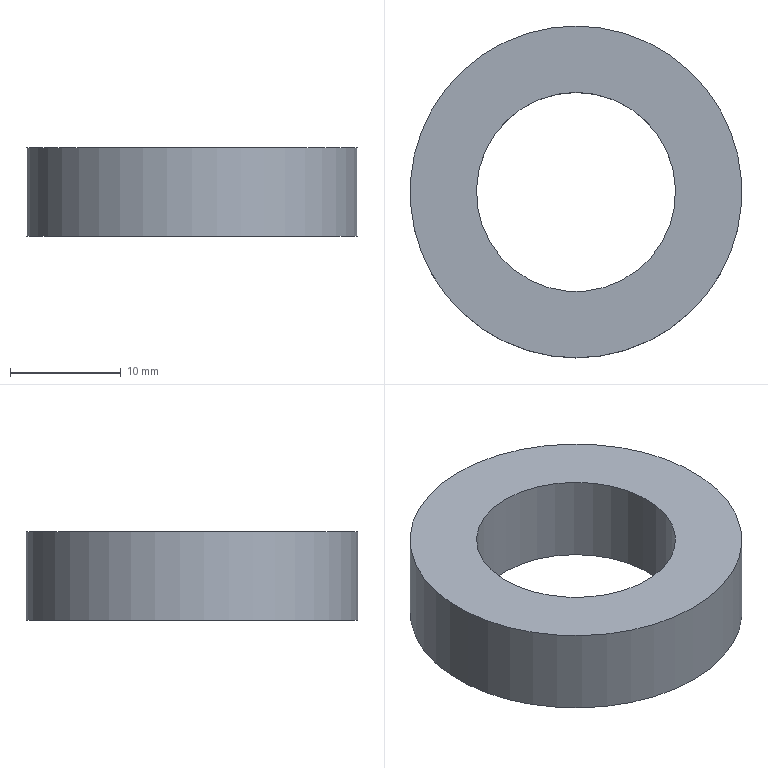Component | NX | 15 | 1 solid | 8 faces | box 30 x 30 x 8 mm | volume 2262 mm3 | plane 4 | cylinder 4 | commonest cylinder face diameters 30 x1 18 x1 21 x1 27 x1
STEP:
#1=CARTESIAN_POINT('',(0.,0.,0.));
#2=DIRECTION('',(0.,0.,1.));
#3=DIRECTION('',(1.,0.,0.));
#4=AXIS2_PLACEMENT_3D('',#1,#2,#3);
#5=CARTESIAN_POINT('',(0.,31.5,-46.));
#6=VERTEX_POINT('',#5);
#7=CARTESIAN_POINT('',(0.,16.5,-46.));
#8=DIRECTION('',(0.,0.,-1.));
#9=DIRECTION('',(0.,1.,0.));
#10=AXIS2_PLACEMENT_3D('',#7,#8,#9);
#11=CIRCLE('',#10,15.);
#12=CARTESIAN_POINT('',(0.,30.,-46.));
#13=DIRECTION('',(0.,0.,-1.));
#14=DIRECTION('',(0.,1.,0.));
#15=AXIS2_PLACEMENT_3D('',#12,#13,#14);
#16=PLANE('',#15);
#17=CARTESIAN_POINT('',(-13.5,0.));
#18=DIRECTION('',(1.,0.));
#19=AXIS2_PLACEMENT_2D('',#17,#18);
#20=CIRCLE('',#19,15.);
#21=(GEOMETRIC_REPRESENTATION_CONTEXT(2)PARAMETRIC_REPRESENTATION_CONTEXT()REPRESENTATION_CONTEXT('',''));
#22=DEFINITIONAL_REPRESENTATION('',(#20),#21);
#23=PCURVE('',#16,#22);
#24=CARTESIAN_POINT('',(0.,16.5,-46.));
#25=DIRECTION('',(0.,0.,-1.));
#26=DIRECTION('',(0.,1.,0.));
#27=AXIS2_PLACEMENT_3D('',#24,#25,#26);
#28=CYLINDRICAL_SURFACE('',#27,15.);
#29=CARTESIAN_POINT('',(0.,0.));
#30=DIRECTION('',(1.,0.));
#31=VECTOR('',#30,1.);
#32=LINE('',#29,#31);
#33=(GEOMETRIC_REPRESENTATION_CONTEXT(2)PARAMETRIC_REPRESENTATION_CONTEXT()REPRESENTATION_CONTEXT('',''));
#34=DEFINITIONAL_REPRESENTATION('',(#32),#33);
#35=PCURVE('',#28,#34);
#36=SURFACE_CURVE('',#11,(#23,#35),.PCURVE_S1.);
#37=EDGE_CURVE('',#6,#6,#36,.T.);
#38=ORIENTED_EDGE('',*,*,#37,.T.);
#39=EDGE_LOOP('',(#38));
#40=FACE_BOUND('',#39,.T.);
#41=CARTESIAN_POINT('',(0.,30.,-46.));
#42=VERTEX_POINT('',#41);
#43=CARTESIAN_POINT('',(0.,16.5,-46.));
#44=DIRECTION('',(0.,0.,-1.));
#45=DIRECTION('',(0.,1.,0.));
#46=AXIS2_PLACEMENT_3D('',#43,#44,#45);
#47=CIRCLE('',#46,13.5);
#48=CARTESIAN_POINT('',(-13.5,0.));
#49=DIRECTION('',(1.,0.));
#50=AXIS2_PLACEMENT_2D('',#48,#49);
#51=CIRCLE('',#50,13.5);
#52=(GEOMETRIC_REPRESENTATION_CONTEXT(2)PARAMETRIC_REPRESENTATION_CONTEXT()REPRESENTATION_CONTEXT('',''));
#53=DEFINITIONAL_REPRESENTATION('',(#51),#52);
#54=PCURVE('',#16,#53);
#55=CARTESIAN_POINT('',(0.,16.5,-46.));
#56=DIRECTION('',(0.,0.,-1.));
#57=DIRECTION('',(0.,1.,0.));
#58=AXIS2_PLACEMENT_3D('',#55,#56,#57);
#59=CYLINDRICAL_SURFACE('',#58,13.5);
#60=CARTESIAN_POINT('',(0.,0.));
#61=DIRECTION('',(1.,0.));
#62=VECTOR('',#61,1.);
#63=LINE('',#60,#62);
#64=(GEOMETRIC_REPRESENTATION_CONTEXT(2)PARAMETRIC_REPRESENTATION_CONTEXT()REPRESENTATION_CONTEXT('',''));
#65=DEFINITIONAL_REPRESENTATION('',(#63),#64);
#66=PCURVE('',#59,#65);
#67=SURFACE_CURVE('',#47,(#54,#66),.PCURVE_S1.);
#68=EDGE_CURVE('',#42,#42,#67,.T.);
#69=ORIENTED_EDGE('',*,*,#68,.F.);
#70=EDGE_LOOP('',(#69));
#71=FACE_BOUND('',#70,.T.);
#72=ADVANCED_FACE('',(#40,#71),#16,.T.);
#73=CARTESIAN_POINT('',(0.,31.5,-38.));
#74=VERTEX_POINT('',#73);
#75=CARTESIAN_POINT('',(0.,16.5,-38.));
#76=DIRECTION('',(0.,0.,-1.));
#77=DIRECTION('',(0.,1.,0.));
#78=AXIS2_PLACEMENT_3D('',#75,#76,#77);
#79=CIRCLE('',#78,15.);
#80=CARTESIAN_POINT('',(0.,-8.));
#81=DIRECTION('',(1.,0.));
#82=VECTOR('',#81,1.);
#83=LINE('',#80,#82);
#84=(GEOMETRIC_REPRESENTATION_CONTEXT(2)PARAMETRIC_REPRESENTATION_CONTEXT()REPRESENTATION_CONTEXT('',''));
#85=DEFINITIONAL_REPRESENTATION('',(#83),#84);
#86=PCURVE('',#28,#85);
#87=CARTESIAN_POINT('',(0.,31.5,-38.));
#88=DIRECTION('',(0.,0.,1.));
#89=DIRECTION('',(0.,-1.,0.));
#90=AXIS2_PLACEMENT_3D('',#87,#88,#89);
#91=PLANE('',#90);
#92=CARTESIAN_POINT('',(0.,0.));
#93=CARTESIAN_POINT('',(0.,25.981));
#94=CARTESIAN_POINT('',(22.5,12.99));
#95=CARTESIAN_POINT('',(45.,0.));
#96=CARTESIAN_POINT('',(22.5,-12.99));
#97=CARTESIAN_POINT('',(0.,-25.981));
#98=CARTESIAN_POINT('',(0.,0.));
#99=(BOUNDED_CURVE()B_SPLINE_CURVE(2,(#92,#93,#94,#95,#96,#97,#98),.UNSPECIFIED.,.T.,.F.)B_SPLINE_CURVE_WITH_KNOTS((1,2,2,2,2,1),(-2.094,0.,2.094,4.189,6.283,8.378),.UNSPECIFIED.)CURVE()GEOMETRIC_REPRESENTATION_ITEM()RATIONAL_B_SPLINE_CURVE((1.,0.5,1.,0.5,1.,0.5,1.))REPRESENTATION_ITEM(''));
#100=(GEOMETRIC_REPRESENTATION_CONTEXT(2)PARAMETRIC_REPRESENTATION_CONTEXT()REPRESENTATION_CONTEXT('',''));
#101=DEFINITIONAL_REPRESENTATION('',(#99),#100);
#102=PCURVE('',#91,#101);
#103=SURFACE_CURVE('',#79,(#86,#102),.PCURVE_S1.);
#104=EDGE_CURVE('',#74,#74,#103,.T.);
#105=ORIENTED_EDGE('',*,*,#104,.T.);
#106=CARTESIAN_POINT('',(0.,31.5,-38.));
#107=CARTESIAN_POINT('',(0.,31.5,-46.));
#108=B_SPLINE_CURVE_WITH_KNOTS('',1,(#106,#107),.UNSPECIFIED.,.F.,.F.,(2,2),(-8.,0.),.PIECEWISE_BEZIER_KNOTS.);
#109=CARTESIAN_POINT('',(6.283,0.));
#110=DIRECTION('',(0.,1.));
#111=VECTOR('',#110,1.);
#112=LINE('',#109,#111);
#113=(GEOMETRIC_REPRESENTATION_CONTEXT(2)PARAMETRIC_REPRESENTATION_CONTEXT()REPRESENTATION_CONTEXT('',''));
#114=DEFINITIONAL_REPRESENTATION('',(#112),#113);
#115=PCURVE('',#28,#114);
#116=CARTESIAN_POINT('',(0.,0.));
#117=DIRECTION('',(0.,1.));
#118=VECTOR('',#117,1.);
#119=LINE('',#116,#118);
#120=(GEOMETRIC_REPRESENTATION_CONTEXT(2)PARAMETRIC_REPRESENTATION_CONTEXT()REPRESENTATION_CONTEXT('',''));
#121=DEFINITIONAL_REPRESENTATION('',(#119),#120);
#122=PCURVE('',#28,#121);
#123=SEAM_CURVE('',#108,(#115,#122),.PCURVE_S1.);
#124=EDGE_CURVE('',#74,#6,#123,.T.);
#125=ORIENTED_EDGE('',*,*,#124,.T.);
#126=ORIENTED_EDGE('',*,*,#37,.F.);
#127=ORIENTED_EDGE('',*,*,#124,.F.);
#128=EDGE_LOOP('',(#105,#125,#126,#127));
#129=FACE_BOUND('',#128,.T.);
#130=ADVANCED_FACE('',(#129),#28,.T.);
#131=CARTESIAN_POINT('',(0.,25.5,-38.));
#132=VERTEX_POINT('',#131);
#133=CARTESIAN_POINT('',(0.,16.5,-38.));
#134=DIRECTION('',(0.,0.,-1.));
#135=DIRECTION('',(0.,1.,0.));
#136=AXIS2_PLACEMENT_3D('',#133,#134,#135);
#137=CIRCLE('',#136,9.);
#138=CARTESIAN_POINT('',(6.,0.));
#139=CARTESIAN_POINT('',(6.,15.588));
#140=CARTESIAN_POINT('',(19.5,7.794));
#141=CARTESIAN_POINT('',(33.,0.));
#142=CARTESIAN_POINT('',(19.5,-7.794));
#143=CARTESIAN_POINT('',(6.,-15.588));
#144=CARTESIAN_POINT('',(6.,0.));
#145=(BOUNDED_CURVE()B_SPLINE_CURVE(2,(#138,#139,#140,#141,#142,#143,#144),.UNSPECIFIED.,.T.,.F.)B_SPLINE_CURVE_WITH_KNOTS((1,2,2,2,2,1),(-2.094,0.,2.094,4.189,6.283,8.378),.UNSPECIFIED.)CURVE()GEOMETRIC_REPRESENTATION_ITEM()RATIONAL_B_SPLINE_CURVE((1.,0.5,1.,0.5,1.,0.5,1.))REPRESENTATION_ITEM(''));
#146=(GEOMETRIC_REPRESENTATION_CONTEXT(2)PARAMETRIC_REPRESENTATION_CONTEXT()REPRESENTATION_CONTEXT('',''));
#147=DEFINITIONAL_REPRESENTATION('',(#145),#146);
#148=PCURVE('',#91,#147);
#149=CARTESIAN_POINT('',(0.,16.5,-46.));
#150=DIRECTION('',(0.,0.,-1.));
#151=DIRECTION('',(0.,1.,0.));
#152=AXIS2_PLACEMENT_3D('',#149,#150,#151);
#153=CYLINDRICAL_SURFACE('',#152,9.);
#154=CARTESIAN_POINT('',(0.,-8.));
#155=DIRECTION('',(1.,0.));
#156=VECTOR('',#155,1.);
#157=LINE('',#154,#156);
#158=(GEOMETRIC_REPRESENTATION_CONTEXT(2)PARAMETRIC_REPRESENTATION_CONTEXT()REPRESENTATION_CONTEXT('',''));
#159=DEFINITIONAL_REPRESENTATION('',(#157),#158);
#160=PCURVE('',#153,#159);
#161=SURFACE_CURVE('',#137,(#148,#160),.PCURVE_S1.);
#162=EDGE_CURVE('',#132,#132,#161,.T.);
#163=ORIENTED_EDGE('',*,*,#162,.T.);
#164=EDGE_LOOP('',(#163));
#165=FACE_BOUND('',#164,.T.);
#166=ORIENTED_EDGE('',*,*,#104,.F.);
#167=EDGE_LOOP('',(#166));
#168=FACE_BOUND('',#167,.T.);
#169=ADVANCED_FACE('',(#165,#168),#91,.T.);
#170=CARTESIAN_POINT('',(0.,25.5,-46.));
#171=VERTEX_POINT('',#170);
#172=CARTESIAN_POINT('',(0.,16.5,-46.));
#173=DIRECTION('',(0.,0.,-1.));
#174=DIRECTION('',(0.,1.,0.));
#175=AXIS2_PLACEMENT_3D('',#172,#173,#174);
#176=CIRCLE('',#175,9.);
#177=CARTESIAN_POINT('',(0.,0.));
#178=DIRECTION('',(1.,0.));
#179=VECTOR('',#178,1.);
#180=LINE('',#177,#179);
#181=(GEOMETRIC_REPRESENTATION_CONTEXT(2)PARAMETRIC_REPRESENTATION_CONTEXT()REPRESENTATION_CONTEXT('',''));
#182=DEFINITIONAL_REPRESENTATION('',(#180),#181);
#183=PCURVE('',#153,#182);
#184=CARTESIAN_POINT('',(0.,25.5,-46.));
#185=DIRECTION('',(0.,0.,-1.));
#186=DIRECTION('',(0.,1.,0.));
#187=AXIS2_PLACEMENT_3D('',#184,#185,#186);
#188=PLANE('',#187);
#189=CARTESIAN_POINT('',(-9.,0.));
#190=DIRECTION('',(1.,0.));
#191=AXIS2_PLACEMENT_2D('',#189,#190);
#192=CIRCLE('',#191,9.);
#193=(GEOMETRIC_REPRESENTATION_CONTEXT(2)PARAMETRIC_REPRESENTATION_CONTEXT()REPRESENTATION_CONTEXT('',''));
#194=DEFINITIONAL_REPRESENTATION('',(#192),#193);
#195=PCURVE('',#188,#194);
#196=SURFACE_CURVE('',#176,(#183,#195),.PCURVE_S1.);
#197=EDGE_CURVE('',#171,#171,#196,.T.);
#198=ORIENTED_EDGE('',*,*,#197,.F.);
#199=CARTESIAN_POINT('',(-0.,25.5,-38.));
#200=CARTESIAN_POINT('',(-0.,25.5,-46.));
#201=B_SPLINE_CURVE_WITH_KNOTS('',1,(#199,#200),.UNSPECIFIED.,.F.,.F.,(2,2),(-8.,0.),.PIECEWISE_BEZIER_KNOTS.);
#202=CARTESIAN_POINT('',(0.,0.));
#203=DIRECTION('',(0.,1.));
#204=VECTOR('',#203,1.);
#205=LINE('',#202,#204);
#206=(GEOMETRIC_REPRESENTATION_CONTEXT(2)PARAMETRIC_REPRESENTATION_CONTEXT()REPRESENTATION_CONTEXT('',''));
#207=DEFINITIONAL_REPRESENTATION('',(#205),#206);
#208=PCURVE('',#153,#207);
#209=CARTESIAN_POINT('',(6.283,0.));
#210=DIRECTION('',(0.,1.));
#211=VECTOR('',#210,1.);
#212=LINE('',#209,#211);
#213=(GEOMETRIC_REPRESENTATION_CONTEXT(2)PARAMETRIC_REPRESENTATION_CONTEXT()REPRESENTATION_CONTEXT('',''));
#214=DEFINITIONAL_REPRESENTATION('',(#212),#213);
#215=PCURVE('',#153,#214);
#216=SEAM_CURVE('',#201,(#208,#215),.PCURVE_S1.);
#217=EDGE_CURVE('',#132,#171,#216,.T.);
#218=ORIENTED_EDGE('',*,*,#217,.F.);
#219=ORIENTED_EDGE('',*,*,#162,.T.);
#220=ORIENTED_EDGE('',*,*,#217,.T.);
#221=EDGE_LOOP('',(#198,#218,#219,#220));
#222=FACE_BOUND('',#221,.F.);
#223=ADVANCED_FACE('',(#222),#153,.F.);
#224=CARTESIAN_POINT('',(0.,27.,-46.));
#225=VERTEX_POINT('',#224);
#226=CARTESIAN_POINT('',(0.,16.5,-46.));
#227=DIRECTION('',(0.,0.,-1.));
#228=DIRECTION('',(0.,1.,0.));
#229=AXIS2_PLACEMENT_3D('',#226,#227,#228);
#230=CIRCLE('',#229,10.5);
#231=CARTESIAN_POINT('',(-9.,0.));
#232=DIRECTION('',(1.,0.));
#233=AXIS2_PLACEMENT_2D('',#231,#232);
#234=CIRCLE('',#233,10.5);
#235=(GEOMETRIC_REPRESENTATION_CONTEXT(2)PARAMETRIC_REPRESENTATION_CONTEXT()REPRESENTATION_CONTEXT('',''));
#236=DEFINITIONAL_REPRESENTATION('',(#234),#235);
#237=PCURVE('',#188,#236);
#238=CARTESIAN_POINT('',(0.,16.5,-46.));
#239=DIRECTION('',(0.,0.,-1.));
#240=DIRECTION('',(0.,1.,0.));
#241=AXIS2_PLACEMENT_3D('',#238,#239,#240);
#242=CYLINDRICAL_SURFACE('',#241,10.5);
#243=CARTESIAN_POINT('',(0.,0.));
#244=DIRECTION('',(1.,0.));
#245=VECTOR('',#244,1.);
#246=LINE('',#243,#245);
#247=(GEOMETRIC_REPRESENTATION_CONTEXT(2)PARAMETRIC_REPRESENTATION_CONTEXT()REPRESENTATION_CONTEXT('',''));
#248=DEFINITIONAL_REPRESENTATION('',(#246),#247);
#249=PCURVE('',#242,#248);
#250=SURFACE_CURVE('',#230,(#237,#249),.PCURVE_S1.);
#251=EDGE_CURVE('',#225,#225,#250,.T.);
#252=ORIENTED_EDGE('',*,*,#251,.T.);
#253=EDGE_LOOP('',(#252));
#254=FACE_BOUND('',#253,.T.);
#255=ORIENTED_EDGE('',*,*,#197,.F.);
#256=EDGE_LOOP('',(#255));
#257=FACE_BOUND('',#256,.T.);
#258=ADVANCED_FACE('',(#254,#257),#188,.T.);
#259=CARTESIAN_POINT('',(0.,27.,-40.));
#260=VERTEX_POINT('',#259);
#261=CARTESIAN_POINT('',(0.,16.5,-40.));
#262=DIRECTION('',(0.,0.,-1.));
#263=DIRECTION('',(0.,1.,0.));
#264=AXIS2_PLACEMENT_3D('',#261,#262,#263);
#265=CIRCLE('',#264,10.5);
#266=CARTESIAN_POINT('',(0.,-6.));
#267=DIRECTION('',(1.,0.));
#268=VECTOR('',#267,1.);
#269=LINE('',#266,#268);
#270=(GEOMETRIC_REPRESENTATION_CONTEXT(2)PARAMETRIC_REPRESENTATION_CONTEXT()REPRESENTATION_CONTEXT('',''));
#271=DEFINITIONAL_REPRESENTATION('',(#269),#270);
#272=PCURVE('',#242,#271);
#273=CARTESIAN_POINT('',(0.,27.,-40.));
#274=DIRECTION('',(0.,0.,-1.));
#275=DIRECTION('',(0.,1.,0.));
#276=AXIS2_PLACEMENT_3D('',#273,#274,#275);
#277=PLANE('',#276);
#278=CARTESIAN_POINT('',(-10.5,0.));
#279=DIRECTION('',(1.,0.));
#280=AXIS2_PLACEMENT_2D('',#278,#279);
#281=CIRCLE('',#280,10.5);
#282=(GEOMETRIC_REPRESENTATION_CONTEXT(2)PARAMETRIC_REPRESENTATION_CONTEXT()REPRESENTATION_CONTEXT('',''));
#283=DEFINITIONAL_REPRESENTATION('',(#281),#282);
#284=PCURVE('',#277,#283);
#285=SURFACE_CURVE('',#265,(#272,#284),.PCURVE_S1.);
#286=EDGE_CURVE('',#260,#260,#285,.T.);
#287=ORIENTED_EDGE('',*,*,#286,.T.);
#288=CARTESIAN_POINT('',(0.,27.,-40.));
#289=CARTESIAN_POINT('',(0.,27.,-46.));
#290=B_SPLINE_CURVE_WITH_KNOTS('',1,(#288,#289),.UNSPECIFIED.,.F.,.F.,(2,2),(-6.,0.),.PIECEWISE_BEZIER_KNOTS.);
#291=CARTESIAN_POINT('',(6.283,0.));
#292=DIRECTION('',(0.,1.));
#293=VECTOR('',#292,1.);
#294=LINE('',#291,#293);
#295=(GEOMETRIC_REPRESENTATION_CONTEXT(2)PARAMETRIC_REPRESENTATION_CONTEXT()REPRESENTATION_CONTEXT('',''));
#296=DEFINITIONAL_REPRESENTATION('',(#294),#295);
#297=PCURVE('',#242,#296);
#298=CARTESIAN_POINT('',(0.,0.));
#299=DIRECTION('',(0.,1.));
#300=VECTOR('',#299,1.);
#301=LINE('',#298,#300);
#302=(GEOMETRIC_REPRESENTATION_CONTEXT(2)PARAMETRIC_REPRESENTATION_CONTEXT()REPRESENTATION_CONTEXT('',''));
#303=DEFINITIONAL_REPRESENTATION('',(#301),#302);
#304=PCURVE('',#242,#303);
#305=SEAM_CURVE('',#290,(#297,#304),.PCURVE_S1.);
#306=EDGE_CURVE('',#260,#225,#305,.T.);
#307=ORIENTED_EDGE('',*,*,#306,.T.);
#308=ORIENTED_EDGE('',*,*,#251,.F.);
#309=ORIENTED_EDGE('',*,*,#306,.F.);
#310=EDGE_LOOP('',(#287,#307,#308,#309));
#311=FACE_BOUND('',#310,.T.);
#312=ADVANCED_FACE('',(#311),#242,.T.);
#313=CARTESIAN_POINT('',(0.,30.,-40.));
#314=VERTEX_POINT('',#313);
#315=CARTESIAN_POINT('',(0.,16.5,-40.));
#316=DIRECTION('',(0.,0.,-1.));
#317=DIRECTION('',(0.,1.,0.));
#318=AXIS2_PLACEMENT_3D('',#315,#316,#317);
#319=CIRCLE('',#318,13.5);
#320=CARTESIAN_POINT('',(-10.5,0.));
#321=DIRECTION('',(1.,0.));
#322=AXIS2_PLACEMENT_2D('',#320,#321);
#323=CIRCLE('',#322,13.5);
#324=(GEOMETRIC_REPRESENTATION_CONTEXT(2)PARAMETRIC_REPRESENTATION_CONTEXT()REPRESENTATION_CONTEXT('',''));
#325=DEFINITIONAL_REPRESENTATION('',(#323),#324);
#326=PCURVE('',#277,#325);
#327=CARTESIAN_POINT('',(0.,-6.));
#328=DIRECTION('',(1.,0.));
#329=VECTOR('',#328,1.);
#330=LINE('',#327,#329);
#331=(GEOMETRIC_REPRESENTATION_CONTEXT(2)PARAMETRIC_REPRESENTATION_CONTEXT()REPRESENTATION_CONTEXT('',''));
#332=DEFINITIONAL_REPRESENTATION('',(#330),#331);
#333=PCURVE('',#59,#332);
#334=SURFACE_CURVE('',#319,(#326,#333),.PCURVE_S1.);
#335=EDGE_CURVE('',#314,#314,#334,.T.);
#336=ORIENTED_EDGE('',*,*,#335,.T.);
#337=EDGE_LOOP('',(#336));
#338=FACE_BOUND('',#337,.T.);
#339=ORIENTED_EDGE('',*,*,#286,.F.);
#340=EDGE_LOOP('',(#339));
#341=FACE_BOUND('',#340,.T.);
#342=ADVANCED_FACE('',(#338,#341),#277,.T.);
#343=ORIENTED_EDGE('',*,*,#68,.F.);
#344=CARTESIAN_POINT('',(-0.,30.,-40.));
#345=CARTESIAN_POINT('',(-0.,30.,-46.));
#346=B_SPLINE_CURVE_WITH_KNOTS('',1,(#344,#345),.UNSPECIFIED.,.F.,.F.,(2,2),(-6.,0.),.PIECEWISE_BEZIER_KNOTS.);
#347=CARTESIAN_POINT('',(0.,0.));
#348=DIRECTION('',(0.,1.));
#349=VECTOR('',#348,1.);
#350=LINE('',#347,#349);
#351=(GEOMETRIC_REPRESENTATION_CONTEXT(2)PARAMETRIC_REPRESENTATION_CONTEXT()REPRESENTATION_CONTEXT('',''));
#352=DEFINITIONAL_REPRESENTATION('',(#350),#351);
#353=PCURVE('',#59,#352);
#354=CARTESIAN_POINT('',(6.283,0.));
#355=DIRECTION('',(0.,1.));
#356=VECTOR('',#355,1.);
#357=LINE('',#354,#356);
#358=(GEOMETRIC_REPRESENTATION_CONTEXT(2)PARAMETRIC_REPRESENTATION_CONTEXT()REPRESENTATION_CONTEXT('',''));
#359=DEFINITIONAL_REPRESENTATION('',(#357),#358);
#360=PCURVE('',#59,#359);
#361=SEAM_CURVE('',#346,(#353,#360),.PCURVE_S1.);
#362=EDGE_CURVE('',#314,#42,#361,.T.);
#363=ORIENTED_EDGE('',*,*,#362,.F.);
#364=ORIENTED_EDGE('',*,*,#335,.T.);
#365=ORIENTED_EDGE('',*,*,#362,.T.);
#366=EDGE_LOOP('',(#343,#363,#364,#365));
#367=FACE_BOUND('',#366,.F.);
#368=ADVANCED_FACE('',(#367),#59,.F.);
#369=CLOSED_SHELL('',(#72,#130,#169,#223,#258,#312,#342,#368));
#370=MANIFOLD_SOLID_BREP('',#369);
#371=(LENGTH_UNIT()NAMED_UNIT(*)SI_UNIT(.MILLI.,.METRE.));
#372=UNCERTAINTY_MEASURE_WITH_UNIT(LENGTH_MEASURE(0.00001),#371,'','');
#373=(NAMED_UNIT(*)PLANE_ANGLE_UNIT()SI_UNIT($,.RADIAN.));
#374=(NAMED_UNIT(*)SI_UNIT($,.STERADIAN.)SOLID_ANGLE_UNIT());
#375=(GEOMETRIC_REPRESENTATION_CONTEXT(3)GLOBAL_UNCERTAINTY_ASSIGNED_CONTEXT((#372))GLOBAL_UNIT_ASSIGNED_CONTEXT((#371,#373,#374))REPRESENTATION_CONTEXT('',''));
#376=ADVANCED_BREP_SHAPE_REPRESENTATION('',(#4,#370),#375);